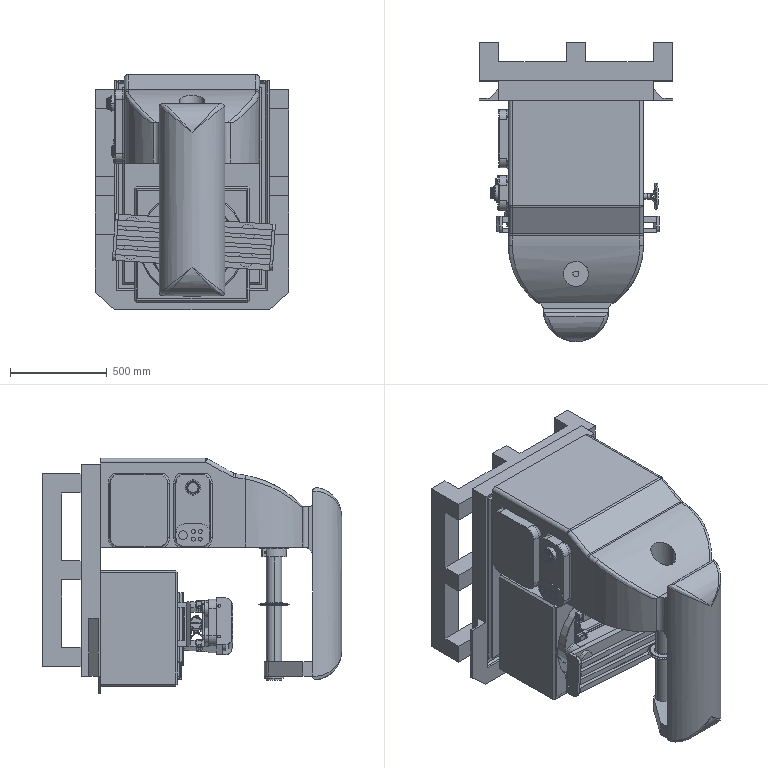Assembly | SolidWorks | mm | 44 component files | 100 solids | 5389 faces | box 1000 x 1550 x 1220 mm | volume 586573695 mm3 | plane 3018 | cylinder 1616 | cone 382 | spline 338 | torus 33 | sphere 2 | commonest cylinder face diameters 0.7 x230 2.8 x132 10.2 x96 20 x94 15 x88 4 x87 1.4 x72 0.28 x56
Bill of materials:
Baffle | 2 |  | Thin flat rectangular plate. The two corners on one long edge are rounded, and two small round through-holes run along the opposite straight edge.
BallScrewPulley | 1 |  | Round handwheel-like part. A rim with a round cross-section connects through four thin straight spokes to a central disc hub. A cylindrical tubular boss sticks out from the hub on one side, and curved webs flare from the boss out to the rim.
BallScrewSupport | 1 |  | T-shaped block bracket. A rectangular plate with two round through-holes has a thick tab sticking out from it. The tab ends in a rounded lug with a larger cross-bore.
Body | 1 |  | Complex bracket or housing with a C-shaped side profile. An upper body with a curved, sloped top and a cross-hole joins a back plate with a flanged, stepped outline. A downward-hanging leg ends in a small cylindrical tip, and a small cylindrical boss with a hole sits inside the C-opening.
Coupling | 1 |  | Plain cylindrical sleeve or tube with a central bore. The bore has a single rectangular keyway slot running along it.
Coupling2 | 1 |  | Cylindrical tubular sleeve with a central through-bore and one rectangular keyway slot in the bore. It looks similar to the other keyed sleeve but with different proportions.
CylinderAxis | 2 |  | Tee-shaped part. A solid cylindrical shaft joins at a right angle to a short cylindrical barrel, and the barrel has a small axial through-hole.
CylinderHousing | 2 |  | Tee-shaped part. A hollow cylindrical tube joins at a right angle to a cylindrical cross barrel, and the barrel has a small axial through-hole.
FixedAxis | 4 |  | Headed cylindrical pin. A straight solid shank has a short flat round head of larger diameter at one end.
GuideRail2 | 2 |  | Long straight bar with a symmetric cross-section that has notches on two opposite faces, giving an H or I shape. A row of six evenly spaced round through-holes runs along its length.
GuideRail | 2 |  | Long straight bar with a cross-section notched on two opposite faces (H or I shape) and small chamfers on some edges. A row of six evenly spaced round through-holes runs along its length.
Housing | 1 |  | Rectangular block with a large circular through-bore taking up most of one face, which makes it a thick-walled square frame. The outer edges have small chamfers.
RetainingRing | 4 |  | Plain annular ring: a short hollow cylinder with a concentric through bore and flat, parallel end faces.
SawBlade | 1 |  | Thin annular disc with many evenly spaced radial slots open at the outer rim, which form tabs around the edge. It has a slightly raised concentric lip around the central bore, and the outer edge tapers to a point in side view.
ServoMotor | 2 |  | Detailed housing with a box-like rectangular body and a square front mounting flange with four corner holes. A cylindrical output shaft with a key slot and an end center hole sticks out from a stepped circular pilot boss. Connector-like housings with angled cylindrical outlets and a covered rectangular boss sit on the top face. Longitudinal grooves run along the body sides.
ToolAxis | 1 |  | Slender solid cylindrical pin with a thin, slightly larger-diameter collar or flange at one end.
ToolHolder | 1 |  | Stepped cylindrical hub. One end face has a small central bore with a keyway notch. A thin outer flange ring sits partway along the length. Below the flange, the short section has an axial slot and small radial holes on flat or recessed areas.
WoodenFrameBase | 1 |  | Rectangular grid frame of square-section bars forming four equal square openings (2x2). Its central and outer bars stand proud on one side, so the edge profiles look comb-like or stepped.
WorkSlat | 4 |  | Long straight prismatic bar of uniform rectangular (near-square) cross-section with flat square-cut ends.
X-AxisBallScrew | 1 |  | Long slender solid round rod. A short band of evenly spaced circumferential grooves or ridges sits near one end, and the rest of the length is plain.
X-AxisBallScrewSupport2 | 1 |  | L-shaped bracket. A flat rectangular mounting plate has two through holes, and a perpendicular boss with a rounded end has a large through bore parallel to the plate.
X-AxisBase | 1 |  | Rectangular plate-like body with thickened flanges along two long edges. Each flange has a row of six small holes or countersunk features. Slotted clip or tab features with small notches stick up near both ends.
X-AxisPedestal | 1 |  | Flat rectangular plate with rounded corners and four through holes, two near each end. A raised rectangular boss on the back carries small hooked snap-tab or clip features near each end.
X-AxisPedestal2 | 1 |  | Flat rectangular plate with four through holes, two near each end. It has small holes on one narrow end edge.
Y-AxisBallScrew | 1 |  | Slender straight solid cylindrical rod with flat ends and a raised helical coil-like ridge wrapped around a middle section of its length; plain cylindrical sections at both ends.
Y-AxisBallScrewSupport | 1 |  | T-section bracket: flat rectangular base plate with two through-holes near opposite ends, and a perpendicular upright web along its center ending in a rounded lobe that has a large through-bore.
Y-AxisBallScrewSupport2 | 1 |  | T-section bracket similar in layout to a flanged clevis: flat rectangular base plate with two through-holes, and a central perpendicular web whose free end is fully rounded and solid (no bore).
Y-AxisBase | 1 |  | Thick circular disc with a stepped side profile; one face has two vertical rows of small holes or dimples near opposite edges, and the other face has rectangular notches/recesses and small raised tabs.
Z-AxisBase | 1 |  | Flanged round body: large chamfered circular flange with a smaller coaxial cylindrical boss on one side; the opposite side has an annular recess around a central tubular hub with a bore. Small thin pin-like protrusions on pads stand up from the flange face next to the boss.
Mates:
1. concentric | Body-1 edge at (0, -400, -300) dir (0, -1, 0) r 150 | Z-AxisBase-2 face at (0, -406, -300) dir (0, 1, 0) r 150
2. coincident | Body-1 face at (-260, -210, -265) dir (-1, 0, 0) | Z-AxisBase-2 face at (-260, -401, -265) dir (-1, 0, 0)
3. concentric | Body-1 face at (-250, -235, -300) dir (-1, 0, 0) r 17.5 | CylinderHousing-2 face at (-250, -235, -300) dir (1, 0, 0) r 25
4. coincident | Body-1 face at (-250, -235, -300) dir (1, 0, 0) | CylinderHousing-2 face at (-250, -235, -300) dir (-1, 0, 0)
5. concentric | Z-AxisBase-2 face at (-200, -376, -300) dir (1, 0, 0) r 17.5 | CylinderAxis-2 face at (-250, -376, -300) dir (1, 0, 0) r 21
6. coincident | Z-AxisBase-2 face at (-250, -376, -300) dir (1, 0, 0) | CylinderAxis-2 face at (-250, -376, -300) dir (-1, 0, 0)
7. concentric | Body-1 edge at (200, -235, -300) dir (1, 0, 0) r 17.5 | CylinderHousing-3 face at (200, -235, -300) dir (1, 0, 0) r 25
8. coincident | Body-1 face at (200, -235, -300) dir (1, 0, 0) | CylinderHousing-3 face at (200, -235, -300) dir (-1, 0, 0)
9. concentric | Z-AxisBase-2 face at (250, -376, -300) dir (1, 0, 0) r 7.5 | CylinderAxis-3 face at (200, -376, -300) dir (1, 0, 0) r 21
10. coincident | Z-AxisBase-2 face at (200, -376, -300) dir (1, 0, 0) | CylinderAxis-3 face at (200, -376, -300) dir (-1, 0, 0)
11. concentric | Y-AxisBase-1 face at (149.094, -601, -164.368) dir (0, -1, 0) r 5.1 | GuideRail-4 face at (149.094, -626, -164.368) dir (0, -1, 0) r 7.5
12. coincident | Y-AxisBase-1 face at (-19.422, -601, -599.371) dir (0, -1, 0) | GuideRail-4 face at (583.692, -601, -339.116) dir (0, 1, 0)
13. concentric | Y-AxisBase-1 face at (129.672, -601, -463.738) dir (0, -1, 0) r 5.1 | GuideRail-4 face at (129.672, -626, -463.738) dir (0, -1, 0) r 7.5
14. coincident | GuideRail-4 face at (136.067, -631, -133.46) dir (-0.9979, 0, 0.06474) | X-AxisBase-2 face at (130.897, -626.5, -213.155) dir (0.9979, 0, -0.06474)
15. coincident | GuideRail-4 face at (583.692, -631, -339.116) dir (0, -1, 0) | X-AxisBase-2 face at (160.834, -631, -215.097) dir (0, 1, 0)
16. width | GuideRail-4 face at (166.004, -631, -135.402) dir (0.06474, 0, 0.9979) | GuideRail-4 face at (142.698, -631, -494.647) dir (-0.06474, 0, -0.9979) | X-AxisBase-2 face at (-166.453, -666, -394.284) dir (-0.06474, 0, -0.9979) | X-AxisBase-2 face at (591.874, -601, -212.999) dir (0.06474, 0, 0.9979)
17. coincident | X-AxisBase-2 face at (591.874, -696, -212.999) dir (0, -1, 0) | GuideRail2-2 face at (-17.932, -696, -634.403) dir (0, 1, 0)
18. coincident | X-AxisBase-2 face at (591.874, -601, -212.999) dir (0.06474, 0, 0.9979) | GuideRail2-2 face at (187.724, -726, -186.779) dir (0.06474, 0, 0.9979)
19. concentric | Z-AxisBase-2 face at (0, -531, -300) dir (0, 1, 0) r 220 | Y-AxisBase-1 face at (0, -541, -300) dir (0, 1, 0) r 220
20. coincident | Z-AxisBase-2 face at (0, -461, -300) dir (0, -1, 0) | Y-AxisBase-1 face at (-19.422, -461, -599.371) dir (0, 1, 0)
21. distance | X-AxisBase-2 face at (185.782, -696, -216.716) dir (0.9979, 0, -0.06474) | GuideRail2-2 face at (217.817, -696, -649.698) dir (0.9979, 0, -0.06474)
22. coincident | GuideRail2-8 face at (-186.12, -721.5, -388.499) dir (-0.06474, 0, -0.9979) | X-AxisPedestal-1 face at (167.379, -706.5, -411.433) dir (0.06474, 0, 0.9979)
23. coincident | GuideRail2-8 face at (19.245, -726, 54.635) dir (0, -1, 0) | X-AxisPedestal-1 face at (167.088, -726, -415.923) dir (0, 1, 0)
24. width | GuideRail2-8 face at (-216.505, -696, 69.93) dir (-0.9979, 0, 0.06474) | GuideRail2-8 face at (262.488, -696, 38.854) dir (0.9979, 0, -0.06474) | X-AxisPedestal-1 face at (166.764, -761, -420.913) dir (0.9979, 0, -0.06474) | X-AxisPedestal-1 face at (-166.797, -696, 307.209) dir (-0.9979, 0, 0.06474)
25. concentric | X-AxisPedestal-1 face at (288.834, -696, -238.433) dir (0, -1, 0) r 25 | X-AxisPedestal2-3 face at (288.834, -831, -238.433) dir (0, 1, 0) r 25
26. concentric | X-AxisPedestal-1 face at (-318.971, -696, -339.295) dir (0, -1, 0) r 25 | X-AxisPedestal2-3 face at (-318.971, -831, -339.295) dir (0, 1, 0) r 25
27. coincident | X-AxisPedestal-1 face at (-166.797, -801, 307.209) dir (0, -1, 0) | X-AxisPedestal2-3 face at (-106.284, -801, 289.801) dir (0, 1, 0)
28. concentric | Baffle-2 face at (403.861, -816, -396.211) dir (0.9979, 0, -0.06474) r 7.5 | X-AxisPedestal2-3 edge at (403.861, -816, -396.211) dir (0.9979, 0, -0.06474) r 7.5
29. concentric | Baffle-2 face at (414.219, -816, -236.546) dir (0.9979, 0, -0.06474) r 7.5 | X-AxisPedestal2-3 face at (394.261, -816, -235.252) dir (0.9979, 0, -0.06474) r 7.5
30. coincident | Baffle-2 face at (414.867, -851, -226.567) dir (-0.9979, 0, 0.06474) | X-AxisPedestal2-3 face at (401.271, -831, -436.127) dir (0.9979, 0, -0.06474)
31. coincident | Baffle-2 face at (414.867, -851, -226.567) dir (-0.9979, 0, 0.06474) | WorkSlat-2 face at (445.832, -816.759, 250.724) dir (0.9979, 0, -0.06474)
32. distance | WorkSlat-2 face at (403.213, -866, -406.19) dir (-0.06474, 0, -0.9979) | Baffle-2 face at (416.24, -801, -437.098) dir (-0.06474, 0, -0.9979)
33. distance | WorkSlat-2 face at (403.213, -886, -406.19) dir (0, -1, 0) | Baffle-2 face at (418.182, -881, -407.161) dir (0, -1, 0)
34. width | X-AxisPedestal-1 face at (-166.797, -696, 307.209) dir (-0.9979, 0, 0.06474) | X-AxisPedestal-1 face at (166.764, -761, -420.913) dir (0.9979, 0, -0.06474) | BallScrewSupport-1 face at (-33.084, -721, -257.632) dir (-0.9979, 0, 0.06474) | BallScrewSupport-1 face at (6.832, -721, -260.222) dir (0.9979, 0, -0.06474)
35. width | X-AxisBase-2 face at (-166.453, -666, -394.284) dir (-0.06474, 0, -0.9979) | X-AxisBase-2 face at (591.874, -601, -212.999) dir (0.06474, 0, 0.9979) | BallScrewSupport-1 face at (6.832, -721, -260.222) dir (0.06474, 0, 0.9979) | BallScrewSupport-1 face at (2.947, -721, -320.096) dir (-0.06474, 0, -0.9979)
36. coincident | X-AxisPedestal-1 face at (-166.797, -731, 307.209) dir (0, 1, 0) | BallScrewSupport-1 face at (552.942, -731, -219.58) dir (0, -1, 0)
37. concentric | BallScrewSupport-1 face at (76.849, -696, -294.827) dir (-0.9979, 0, 0.06474) r 10 | X-AxisBallScrew-2 face at (50.551, -696, -293.121) dir (-0.9979, 0, 0.06474) r 10
38. width | X-AxisBallScrew-2 plane at (96.342, -353.787, 412.691) dir (0.9979, 0, -0.06474) | X-AxisBallScrew-2 plane at (-3.448, -353.787, 419.165) dir (-0.9979, 0, 0.06474) | X-AxisBase-2 face at (-166.453, -666, -394.284) dir (-0.9979, 0, 0.06474) | X-AxisBase-2 face at (165.824, -636, -215.421) dir (0.9979, 0, -0.06474)
39. concentric | X-AxisBallScrew-2 face at (50.551, -696, -293.121) dir (-0.9979, 0, 0.06474) r 10 | ServoMotor-1 face at (-127.375, -696, -281.578) dir (-0.9979, 0, 0.06474) r 6.65
40. concentric | ServoMotor-1 face at (-127.375, -696, -281.578) dir (-0.9979, 0, 0.06474) r 6.65 | Coupling-1 face at (-149.029, -696, -280.173) dir (0.9979, 0, -0.06474) r 6.65
41. parallel | X-AxisPedestal-1 face at (-166.797, -731, 307.209) dir (0, 1, 0) | ServoMotor-1 face at (-236.303, -724, -256.915) dir (0, -1, 0)
42. coincident | ServoMotor-1 face at (-149.925, -709.832, -293.989) dir (0.9979, 0, -0.06474) | Coupling-1 face at (-149.029, -696, -280.173) dir (-0.9979, 0, 0.06474)
43. distance | Coupling-1 face at (-89.155, -696, -284.058) dir (0.9979, 0, -0.06474) | X-AxisBallScrew-2 face at (-109.113, -696, -282.763) dir (-0.9979, 0, 0.06474)
44. coincident | X-AxisBase-2 face at (591.874, -666, -212.999) dir (0, -1, 0) | X-AxisBallScrewSupport2-2 face at (178.042, -666, 436.306) dir (0, 1, 0)
45. concentric | X-AxisBallScrew-2 face at (50.551, -696, -293.121) dir (-0.9979, 0, 0.06474) r 10 | X-AxisBallScrewSupport2-2 face at (130.384, -696, -298.3) dir (0.9979, 0, -0.06474) r 10
46. coincident | Y-AxisBase-1 face at (0, -551, -300) dir (0, -1, 0) | Y-AxisBallScrewSupport2-1 face at (-729.104, -551, -167.52) dir (0, 1, 0)
47. coincident | X-AxisBase-2 face at (591.874, -636, -212.999) dir (0, 1, 0) | Y-AxisBallScrewSupport-1 face at (-68.627, -636, 278.126) dir (0, -1, 0)
48. width | Y-AxisBallScrewSupport-1 face at (-30.576, -626, -307.9) dir (-0.06474, 0, -0.9979) | Y-AxisBallScrewSupport-1 face at (-27.986, -626, -267.984) dir (0.06474, 0, 0.9979) | X-AxisBase-2 face at (-166.453, -666, -394.284) dir (-0.06474, 0, -0.9979) | X-AxisBase-2 face at (591.874, -601, -212.999) dir (0.06474, 0, 0.9979)
49. width | Y-AxisBallScrewSupport-1 face at (31.888, -626, -271.868) dir (0.9979, 0, -0.06474) | Y-AxisBallScrewSupport-1 face at (-27.986, -626, -267.984) dir (-0.9979, 0, 0.06474) | X-AxisBase-2 face at (165.824, -636, -215.421) dir (0.9979, 0, -0.06474) | X-AxisBase-2 face at (-166.453, -666, -394.284) dir (-0.9979, 0, 0.06474)
50. concentric | Y-AxisBallScrewSupport-1 face at (7.007, -591, -191.987) dir (-0.06474, 0, -0.9979) r 15 | Y-AxisBallScrewSupport2-1 face at (5.503, -591, -215.178) dir (0.06474, 0, 0.9979) r 10
51. concentric | Y-AxisBallScrewSupport-1 face at (7.007, -591, -191.987) dir (-0.06474, 0, -0.9979) r 10 | Y-AxisBallScrew-1 face at (-4.532, -591, -369.853) dir (0.06474, 0, 0.9979) r 10
52. coincident | Y-AxisBallScrewSupport2-1 face at (7.121, -591, -190.231) dir (-0.06474, 0, -0.9979) | Y-AxisBallScrew-1 face at (7.121, -591, -190.231) dir (0.06474, 0, 0.9979)
53. concentric | Coupling2-1 face at (-10.358, -591, -459.664) dir (0.06474, 0, 0.9979) r 6.65 | ServoMotor-2 face at (-8.954, -591, -438.01) dir (-0.06474, 0, -0.9979) r 6.65
54. coincident | Coupling2-1 face at (-10.358, -591, -459.664) dir (-0.06474, 0, -0.9979) | ServoMotor-2 face at (-24.175, -577.168, -458.768) dir (0.06474, 0, 0.9979)
55. concentric | Y-AxisBallScrew-1 face at (-4.532, -591, -369.853) dir (0.06474, 0, 0.9979) r 10 | ServoMotor-2 face at (-8.954, -591, -438.01) dir (-0.06474, 0, -0.9979) r 6.65
56. parallel | Y-AxisBase-1 face at (0, -551, -300) dir (0, -1, 0) | ServoMotor-2 face at (1.428, -563, -549.211) dir (0, 1, 0)
57. distance | Coupling2-1 face at (-6.474, -591, -399.79) dir (0.06474, 0, 0.9979) | Y-AxisBallScrew-1 face at (-7.769, -591, -419.748) dir (-0.06474, 0, -0.9979)
58. concentric | CylinderHousing-2 face at (-225, -335, -300) dir (0, 1, 0) r 25 | CylinderAxis-2 face at (-225, -265, -300) dir (0, -1, 0) r 21
59. distance | CylinderAxis-2 face at (-225, -265, -300) dir (0, 1, 0) | CylinderHousing-2 face at (-225, -265, -300) dir (0, -1, 0)
60. width | Y-AxisBallScrew-1 face at (-7.769, -591, -419.748) dir (-0.06474, 0, -0.9979) | Y-AxisBallScrew-1 face at (7.121, -591, -190.231) dir (0.06474, 0, 0.9979) | GuideRail-5 face at (-143.345, -631, -115.332) dir (0.06474, 0, 0.9979) | GuideRail-5 face at (-166.652, -631, -474.577) dir (-0.06474, 0, -0.9979)
61. concentric | Body-1 face at (0, -1100, 550) dir (0, 0, -1) r 65 | ToolHolder-2 face at (0, -1100, 220) dir (0, 0, -1) r 65
62. coincident | Body-1 face at (-350, -1250, 120) dir (0, 0, -1) | ToolHolder-2 face at (896.819, -1175.599, 120) dir (0, 0, 1)
63. concentric | CylinderHousing-3 face at (225, -335, -300) dir (0, 1, 0) r 25 | CylinderAxis-3 face at (225, -265, -300) dir (0, -1, 0) r 21
64. coincident | X-AxisBallScrew-2 face at (369.88, -696, -313.838) dir (0.9979, 0, -0.06474) | BallScrewPulley-1 face at (369.88, -696, -313.838) dir (-0.9979, 0, 0.06474)
65. concentric | X-AxisBallScrew-2 face at (50.551, -696, -293.121) dir (-0.9979, 0, 0.06474) r 10 | BallScrewPulley-1 face at (339.943, -696, -311.896) dir (0.9979, 0, -0.06474) r 15
66. concentric | ToolAxis-1 face at (0, -1100, -570) dir (0, 0, 1) r 40 | SawBlade-1 face at (0, -1100, -181.726) dir (0, 0, 1) r 40
67. width | Body-1 face at (-170, -1250, -473.452) dir (0, 0, 1) | Body-1 face at (-350, -1250, 120) dir (0, 0, -1) | SawBlade-1 face at (0, -1100, -181.726) dir (0, 0, -1) | SawBlade-1 face at (0, -1100, -171.726) dir (0, 0, 1)
68. concentric | Body-1 face at (0, -1100, -78.991) dir (0, 0, -1) r 40 | ToolAxis-1 face at (0, -1100, -570) dir (0, 0, 1) r 40
69. coincident | Body-1 face at (0, -200, 0) dir (0, -1, 0) | Housing-1 face at (-0.7059, -200, -106.49) dir (0, 1, 0)
70. width | Body-1 face at (400, -200, -550) dir (1, 0, 0) | Body-1 face at (-400, -200, -550) dir (-1, 0, 0) | Housing-1 face at (-300, -600, -600) dir (-1, 0, 0) | Housing-1 face at (300, -600, -600) dir (1, 0, 0)
71. distance | Body-1 face at (-400, -190, -640) dir (0, 0, -1) | Housing-1 face at (300, -600, -600) dir (0, 0, -1)
72. concentric | X-AxisPedestal-1 face at (-318.971, -696, -339.295) dir (0, -1, 0) r 25 | FixedAxis-2 face at (-318.971, -731, -339.295) dir (0, -1, 0) r 25
73. coincident | X-AxisPedestal2-3 face at (-106.284, -831, 289.801) dir (0, -1, 0) | FixedAxis-2 face at (-318.971, -831, -339.295) dir (0, 1, 0)
74. concentric | FixedAxis-2 face at (-318.971, -731, -339.295) dir (0, -1, 0) r 25 | RetainingRing-2 face at (-318.971, -741, -339.295) dir (0, -1, 0) r 25
75. coincident | X-AxisPedestal-1 face at (-166.797, -761, 307.209) dir (0, 1, 0) | RetainingRing-2 face at (-318.971, -761, -339.295) dir (0, -1, 0)
76. concentric | FixedAxis-3 face at (279.77, -731, -378.139) dir (0, -1, 0) r 25 | RetainingRing-3 face at (279.77, -741, -378.139) dir (0, -1, 0) r 25
77. concentric | X-AxisPedestal2-3 face at (279.77, -831, -378.139) dir (0, 1, 0) r 25 | FixedAxis-3 face at (279.77, -731, -378.139) dir (0, -1, 0) r 25
78. coincident | X-AxisPedestal2-3 face at (-106.284, -831, 289.801) dir (0, -1, 0) | FixedAxis-3 face at (279.77, -831, -378.139) dir (0, 1, 0)
79. coincident | X-AxisPedestal-1 face at (-166.797, -761, 307.209) dir (0, 1, 0) | RetainingRing-3 face at (279.77, -761, -378.139) dir (0, -1, 0)
80. concentric | FixedAxis-5 face at (288.834, -731, -238.433) dir (0, -1, 0) r 25 | RetainingRing-5 face at (288.834, -741, -238.433) dir (0, -1, 0) r 25
81. concentric | X-AxisPedestal2-3 edge at (288.834, -831, -238.433) dir (0, 1, 0) r 25 | FixedAxis-5 face at (288.834, -731, -238.433) dir (0, -1, 0) r 25
82. coincident | X-AxisPedestal2-3 face at (-106.284, -831, 289.801) dir (0, -1, 0) | FixedAxis-5 face at (288.834, -831, -238.433) dir (0, 1, 0)
83. coincident | X-AxisPedestal-1 face at (-166.797, -761, 307.209) dir (0, 1, 0) | RetainingRing-5 face at (288.834, -761, -238.433) dir (0, -1, 0)
84. concentric | FixedAxis-7 face at (-309.907, -731, -199.589) dir (0, -1, 0) r 25 | RetainingRing-7 face at (-309.907, -741, -199.589) dir (0, -1, 0) r 25
85. concentric | X-AxisPedestal2-3 face at (-309.907, -831, -199.589) dir (0, 1, 0) r 25 | FixedAxis-7 face at (-309.907, -731, -199.589) dir (0, -1, 0) r 25
86. coincident | X-AxisPedestal2-3 face at (-106.284, -831, 289.801) dir (0, -1, 0) | FixedAxis-7 face at (-309.907, -831, -199.589) dir (0, 1, 0)
87. coincident | X-AxisPedestal-1 face at (-166.797, -761, 307.209) dir (0, 1, 0) | RetainingRing-7 face at (-309.907, -761, -199.589) dir (0, -1, 0)
88. coincident | X-AxisBase-2 face at (165.824, -636, -215.421) dir (0.9979, 0, -0.06474) | X-AxisBallScrewSupport2-2 face at (207.979, -970.698, 434.364) dir (0.9979, 0, -0.06474)